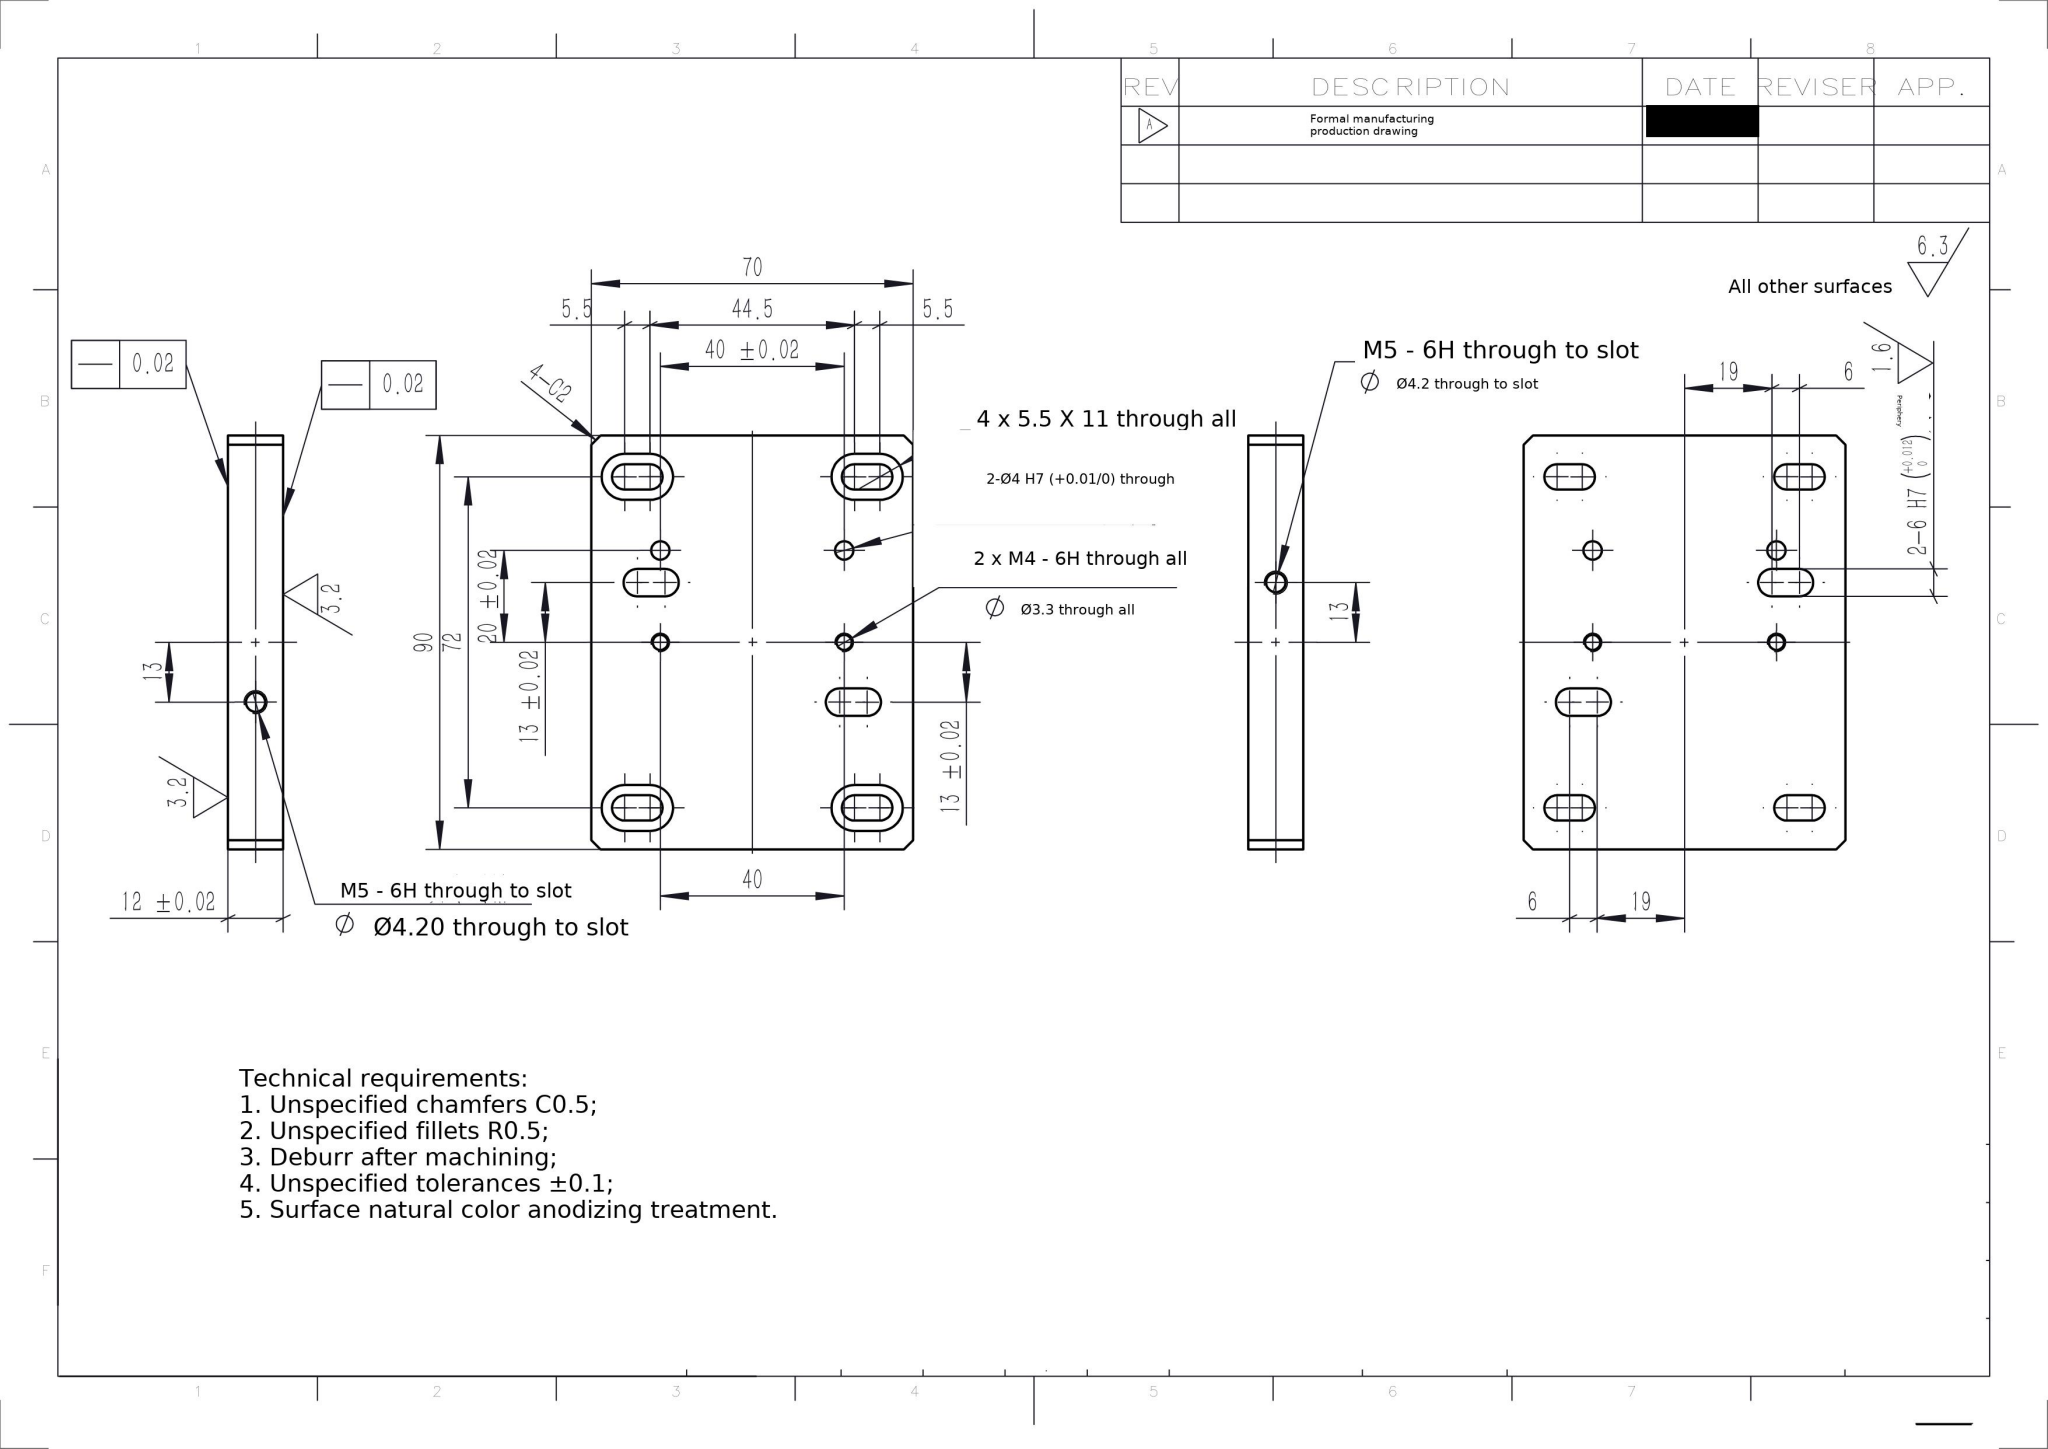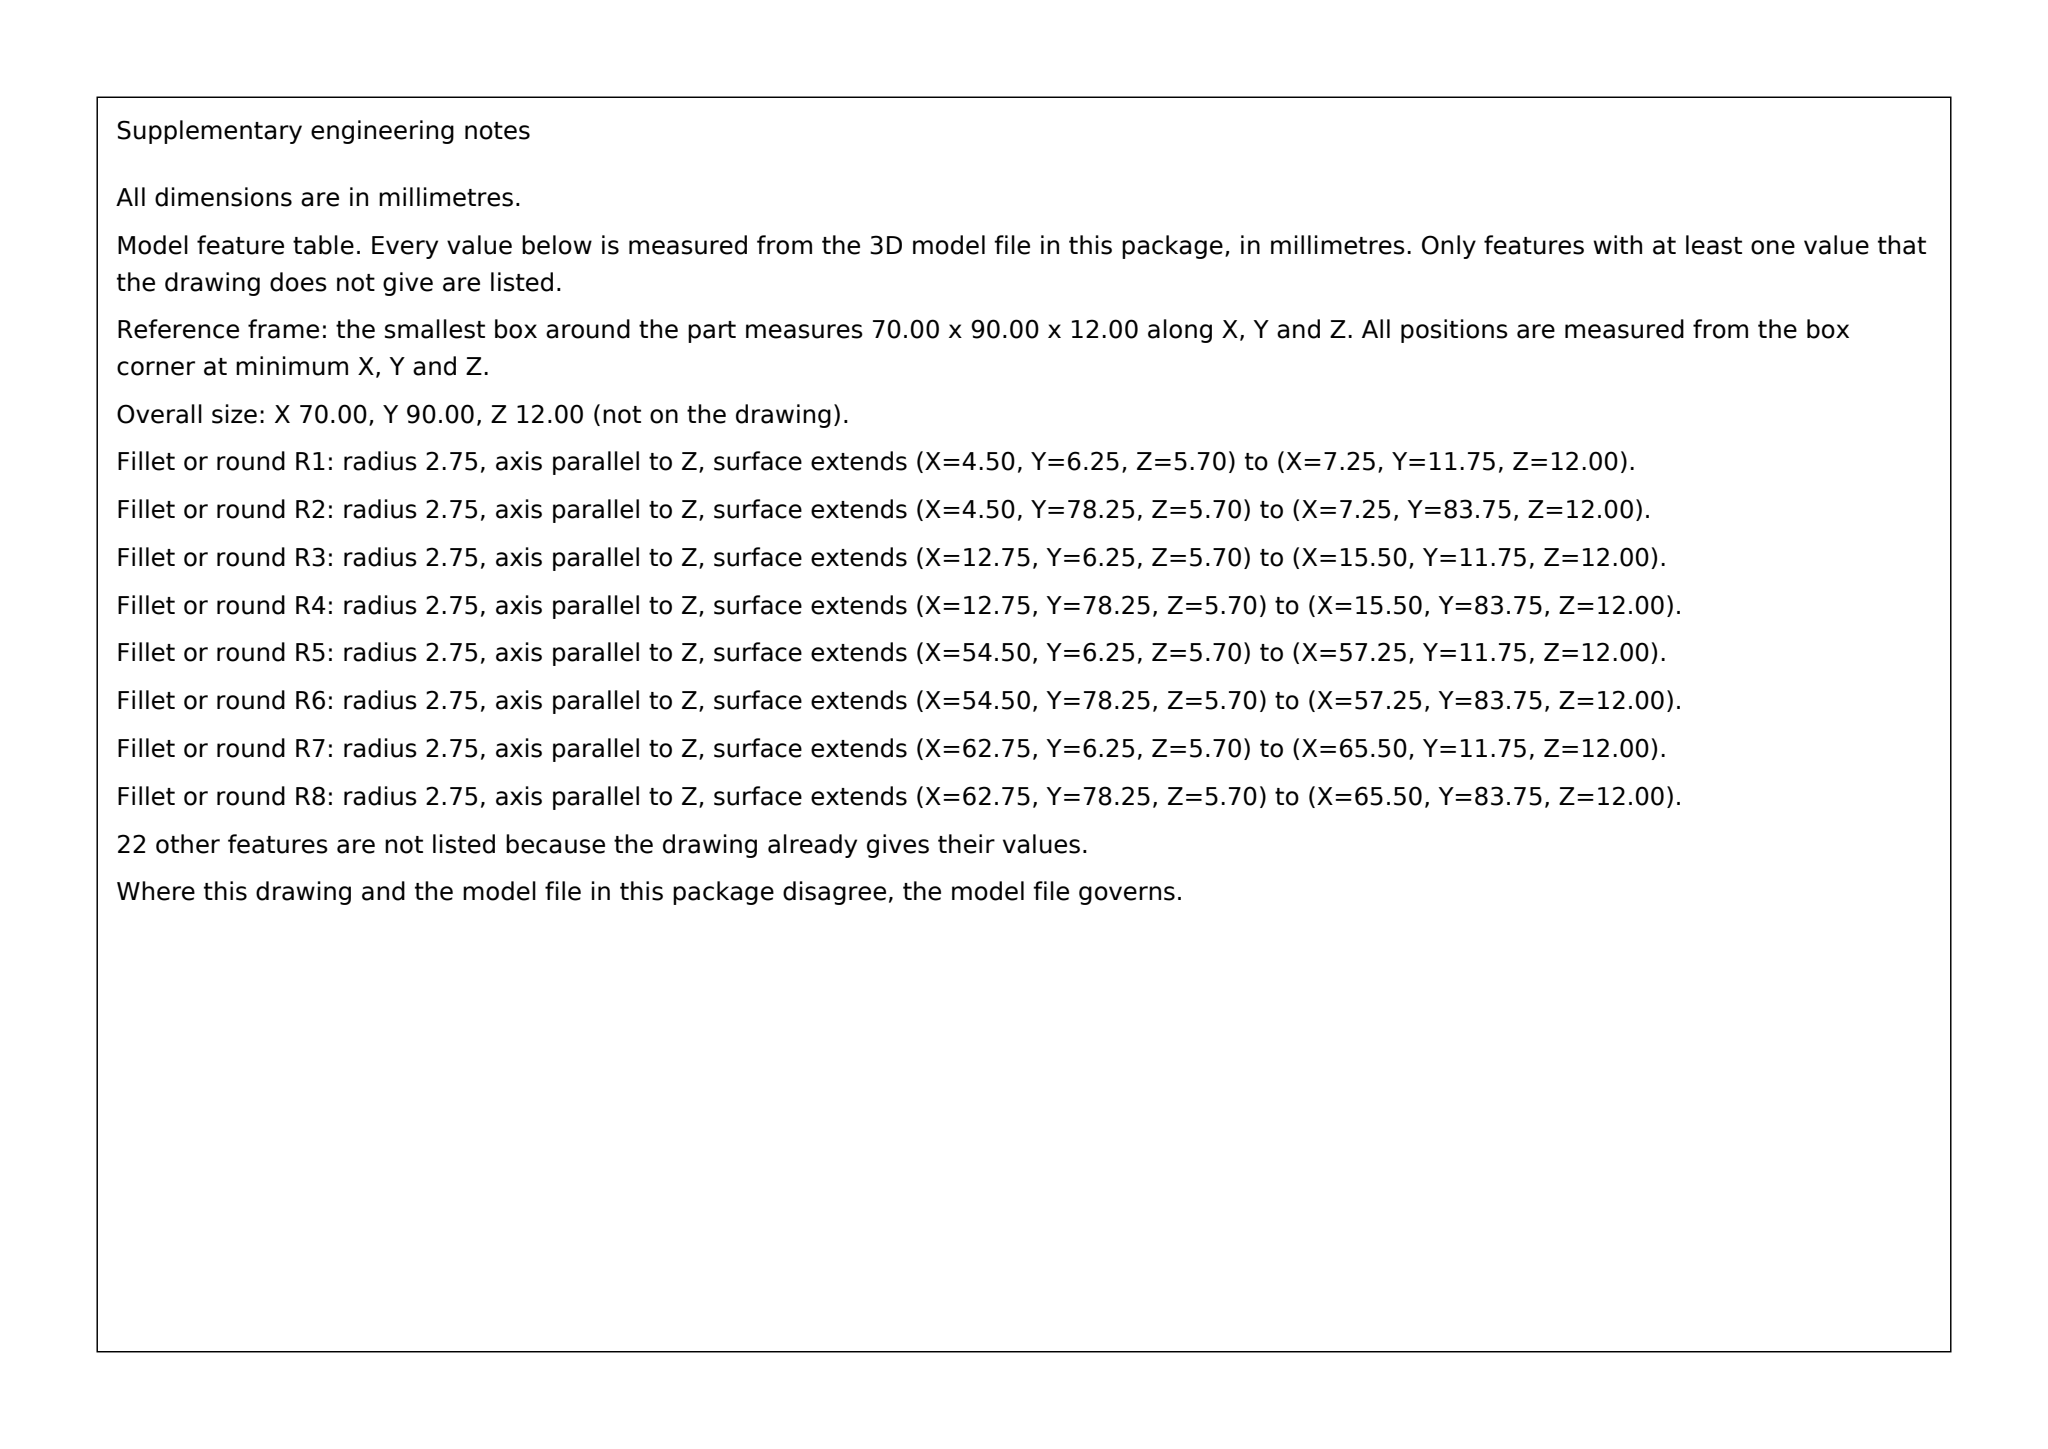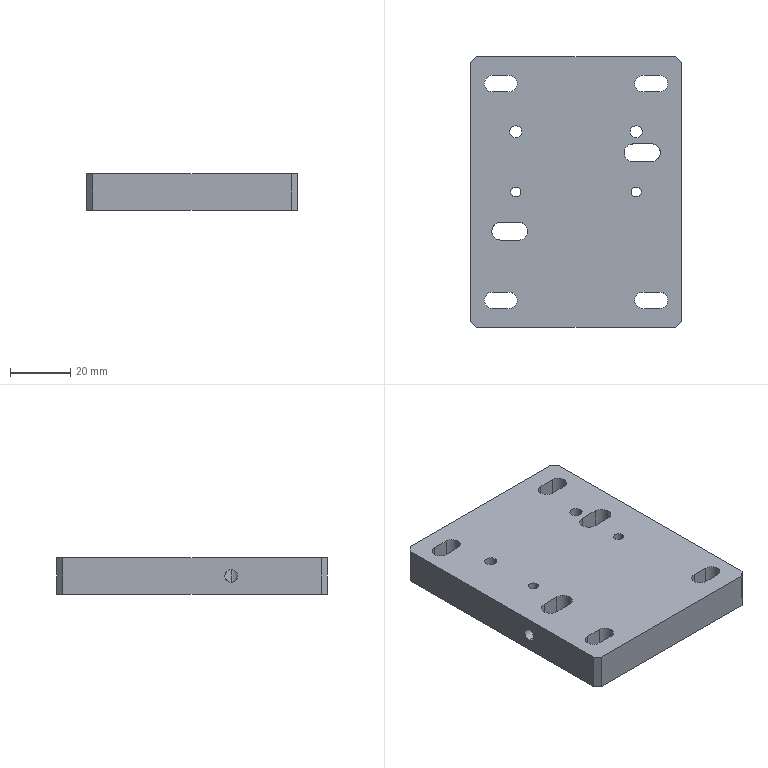Part | SolidWorks | mm | 1 solid | 76 faces | box 70 x 90 x 12 mm | volume 68849 mm3 | cylinder 42 | plane 34 | commonest cylinder face diameters 10 x12 5.5 x12 6 x6 4.2 x4 4 x4 3.3 x4